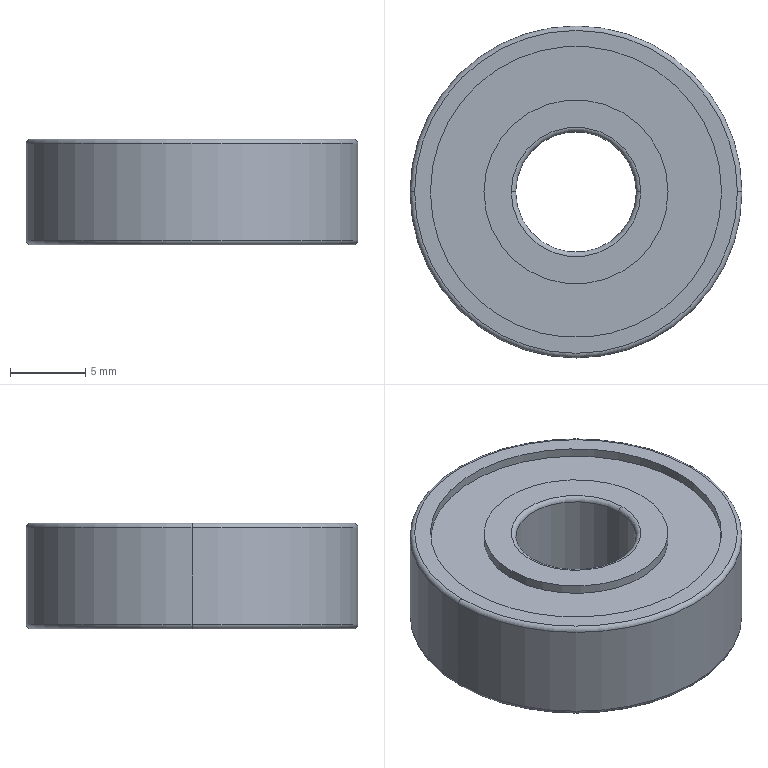Component | SolidWorks | JL001-05-02-1_B608ZZ-1 | 1 solid | 26 faces | box 22 x 22 x 7 mm | volume 2095 mm3 | cylinder 12 | torus 8 | plane 6 | commonest cylinder face diameters 12.2 x4 19.3 x4 22 x2 8 x2
build123d program:
from build123d import *


with BuildPart() as part:
    # Sketch1 → Revolve1 (revolve)
    with BuildSketch(Plane.XY, mode=Mode.PRIVATE) as revolve1_sk:
        with BuildLine():
            Line((0.3, 4), (6.7, 4))
            ThreePointArc((6.7, 4), (6.912, 4.088), (7, 4.3))
            Line((7, 4.3), (7, 6.1))
            Line((7, 6.1), (6.4, 6.1))
            Line((6.4, 6.1), (6.4, 9.65))
            Line((6.4, 9.65), (7, 9.65))
            Line((7, 9.65), (7, 10.7))
            ThreePointArc((7, 10.7), (6.912, 10.912), (6.7, 11))
            Line((6.7, 11), (0.3, 11))
            ThreePointArc((0.3, 11), (0.08787, 10.912), (0, 10.7))
            Line((0, 10.7), (0, 9.65))
            Line((0, 9.65), (0.6, 9.65))
            Line((0.6, 9.65), (0.6, 6.1))
            Line((0.6, 6.1), (0, 6.1))
            Line((0, 6.1), (0, 4.3))
            ThreePointArc((0, 4.3), (0.08787, 4.088), (0.3, 4))
        make_face()
    revolve(revolve1_sk.sketch.rotate(Axis((6.7, 0, 0), (-1, 0, 0)), 270), axis=Axis((6.7, 0, 0), (-1, 0, 0)))


solid = part.part

# Placed as in the assembly
solid = solid.moved(Location((0, 1047.5, 88), (0, 90, 0)))
STEP:
#1=COLOUR_RGB('',0.7922,0.8196,0.9333);
#2=FILL_AREA_STYLE_COLOUR('',#1);
#3=FILL_AREA_STYLE('',(#2));
#4=SURFACE_STYLE_FILL_AREA(#3);
#5=SURFACE_SIDE_STYLE('',(#4));
#6=SURFACE_STYLE_USAGE(.BOTH.,#5);
#7=PRESENTATION_STYLE_ASSIGNMENT((#6));
#8=CARTESIAN_POINT('',(-0.2402,41.24,3.441));
#9=VERTEX_POINT('',#8);
#10=CARTESIAN_POINT('',(0.2402,41.24,3.441));
#11=VERTEX_POINT('',#10);
#12=CARTESIAN_POINT('',(-0.,41.24,3.441));
#13=DIRECTION('',(0.,0.,1.));
#14=DIRECTION('',(-1.,0.,0.));
#15=AXIS2_PLACEMENT_3D('',#12,#13,#14);
#16=CIRCLE('',#15,0.2402);
#17=EDGE_CURVE('',#9,#11,#16,.T.);
#18=ORIENTED_EDGE('',*,*,#17,.T.);
#19=CARTESIAN_POINT('',(0.2402,41.24,3.465));
#20=VERTEX_POINT('',#19);
#21=CARTESIAN_POINT('',(0.2402,41.24,3.201));
#22=DIRECTION('',(0.,0.,1.));
#23=VECTOR('',#22,39.37);
#24=LINE('',#21,#23);
#25=EDGE_CURVE('',#11,#20,#24,.T.);
#26=ORIENTED_EDGE('',*,*,#25,.T.);
#27=CARTESIAN_POINT('',(-0.2402,41.24,3.465));
#28=VERTEX_POINT('',#27);
#29=CARTESIAN_POINT('',(-0.,41.24,3.465));
#30=DIRECTION('',(0.,0.,1.));
#31=DIRECTION('',(-1.,0.,0.));
#32=AXIS2_PLACEMENT_3D('',#29,#30,#31);
#33=CIRCLE('',#32,0.2402);
#34=EDGE_CURVE('',#28,#20,#33,.T.);
#35=ORIENTED_EDGE('',*,*,#34,.F.);
#36=CARTESIAN_POINT('',(-0.2402,41.24,3.201));
#37=DIRECTION('',(0.,0.,1.));
#38=VECTOR('',#37,39.37);
#39=LINE('',#36,#38);
#40=EDGE_CURVE('',#9,#28,#39,.T.);
#41=ORIENTED_EDGE('',*,*,#40,.F.);
#42=EDGE_LOOP('',(#18,#26,#35,#41));
#43=FACE_OUTER_BOUND('',#42,.T.);
#44=CARTESIAN_POINT('',(-0.,41.24,3.201));
#45=DIRECTION('',(0.,0.,1.));
#46=DIRECTION('',(-1.,0.,0.));
#47=AXIS2_PLACEMENT_3D('',#44,#45,#46);
#48=CYLINDRICAL_SURFACE('',#47,0.2402);
#49=ADVANCED_FACE('',(#43),#48,.T.);
#50=CARTESIAN_POINT('',(0.3799,41.24,3.441));
#51=VERTEX_POINT('',#50);
#52=CARTESIAN_POINT('',(-0.3799,41.24,3.441));
#53=VERTEX_POINT('',#52);
#54=CARTESIAN_POINT('',(-0.,41.24,3.441));
#55=DIRECTION('',(0.,0.,1.));
#56=DIRECTION('',(-1.,0.,0.));
#57=AXIS2_PLACEMENT_3D('',#54,#55,#56);
#58=CIRCLE('',#57,0.3799);
#59=EDGE_CURVE('',#51,#53,#58,.T.);
#60=ORIENTED_EDGE('',*,*,#59,.F.);
#61=CARTESIAN_POINT('',(0.3799,41.24,3.465));
#62=VERTEX_POINT('',#61);
#63=CARTESIAN_POINT('',(0.3799,41.24,3.201));
#64=DIRECTION('',(0.,0.,1.));
#65=VECTOR('',#64,39.37);
#66=LINE('',#63,#65);
#67=EDGE_CURVE('',#51,#62,#66,.T.);
#68=ORIENTED_EDGE('',*,*,#67,.T.);
#69=CARTESIAN_POINT('',(-0.3799,41.24,3.465));
#70=VERTEX_POINT('',#69);
#71=CARTESIAN_POINT('',(-0.,41.24,3.465));
#72=DIRECTION('',(0.,0.,1.));
#73=DIRECTION('',(-1.,0.,0.));
#74=AXIS2_PLACEMENT_3D('',#71,#72,#73);
#75=CIRCLE('',#74,0.3799);
#76=EDGE_CURVE('',#62,#70,#75,.T.);
#77=ORIENTED_EDGE('',*,*,#76,.T.);
#78=CARTESIAN_POINT('',(-0.3799,41.24,3.201));
#79=DIRECTION('',(0.,0.,1.));
#80=VECTOR('',#79,39.37);
#81=LINE('',#78,#80);
#82=EDGE_CURVE('',#53,#70,#81,.T.);
#83=ORIENTED_EDGE('',*,*,#82,.F.);
#84=EDGE_LOOP('',(#60,#68,#77,#83));
#85=FACE_OUTER_BOUND('',#84,.T.);
#86=CARTESIAN_POINT('',(-0.,41.24,3.201));
#87=DIRECTION('',(0.,0.,1.));
#88=DIRECTION('',(-1.,0.,0.));
#89=AXIS2_PLACEMENT_3D('',#86,#87,#88);
#90=CYLINDRICAL_SURFACE('',#89,0.3799);
#91=ADVANCED_FACE('',(#85),#90,.F.);
#92=CARTESIAN_POINT('',(-0.4331,41.24,3.453));
#93=VERTEX_POINT('',#92);
#94=CARTESIAN_POINT('',(0.4331,41.24,3.453));
#95=VERTEX_POINT('',#94);
#96=CARTESIAN_POINT('',(-0.,41.24,3.453));
#97=DIRECTION('',(0.,0.,1.));
#98=DIRECTION('',(-1.,0.,0.));
#99=AXIS2_PLACEMENT_3D('',#96,#97,#98);
#100=CIRCLE('',#99,0.4331);
#101=EDGE_CURVE('',#93,#95,#100,.T.);
#102=ORIENTED_EDGE('',*,*,#101,.T.);
#103=CARTESIAN_POINT('',(0.4213,41.24,3.465));
#104=VERTEX_POINT('',#103);
#105=CARTESIAN_POINT('',(0.4213,41.24,3.453));
#106=DIRECTION('',(-0.,-1.,0.));
#107=DIRECTION('',(1.,0.,0.));
#108=AXIS2_PLACEMENT_3D('',#105,#106,#107);
#109=CIRCLE('',#108,0.01181);
#110=EDGE_CURVE('',#95,#104,#109,.T.);
#111=ORIENTED_EDGE('',*,*,#110,.T.);
#112=CARTESIAN_POINT('',(-0.4213,41.24,3.465));
#113=VERTEX_POINT('',#112);
#114=CARTESIAN_POINT('',(-0.,41.24,3.465));
#115=DIRECTION('',(0.,0.,1.));
#116=DIRECTION('',(-1.,0.,0.));
#117=AXIS2_PLACEMENT_3D('',#114,#115,#116);
#118=CIRCLE('',#117,0.4213);
#119=EDGE_CURVE('',#113,#104,#118,.T.);
#120=ORIENTED_EDGE('',*,*,#119,.F.);
#121=CARTESIAN_POINT('',(-0.4213,41.24,3.453));
#122=DIRECTION('',(0.,1.,0.));
#123=DIRECTION('',(0.,0.,1.));
#124=AXIS2_PLACEMENT_3D('',#121,#122,#123);
#125=CIRCLE('',#124,0.01181);
#126=EDGE_CURVE('',#93,#113,#125,.T.);
#127=ORIENTED_EDGE('',*,*,#126,.F.);
#128=EDGE_LOOP('',(#102,#111,#120,#127));
#129=FACE_OUTER_BOUND('',#128,.T.);
#130=CARTESIAN_POINT('',(-0.,41.24,3.453));
#131=DIRECTION('',(0.,0.,1.));
#132=DIRECTION('',(-1.,0.,0.));
#133=AXIS2_PLACEMENT_3D('',#130,#131,#132);
#134=TOROIDAL_SURFACE('',#133,0.4213,0.01181);
#135=ADVANCED_FACE('',(#129),#134,.T.);
#136=CARTESIAN_POINT('',(-0.4331,41.24,3.201));
#137=VERTEX_POINT('',#136);
#138=CARTESIAN_POINT('',(0.4331,41.24,3.201));
#139=VERTEX_POINT('',#138);
#140=CARTESIAN_POINT('',(-0.,41.24,3.201));
#141=DIRECTION('',(0.,0.,1.));
#142=DIRECTION('',(-1.,0.,0.));
#143=AXIS2_PLACEMENT_3D('',#140,#141,#142);
#144=CIRCLE('',#143,0.4331);
#145=EDGE_CURVE('',#137,#139,#144,.T.);
#146=ORIENTED_EDGE('',*,*,#145,.T.);
#147=CARTESIAN_POINT('',(0.4331,41.24,3.201));
#148=DIRECTION('',(0.,0.,1.));
#149=VECTOR('',#148,39.37);
#150=LINE('',#147,#149);
#151=EDGE_CURVE('',#139,#95,#150,.T.);
#152=ORIENTED_EDGE('',*,*,#151,.T.);
#153=ORIENTED_EDGE('',*,*,#101,.F.);
#154=CARTESIAN_POINT('',(-0.4331,41.24,3.201));
#155=DIRECTION('',(0.,0.,1.));
#156=VECTOR('',#155,39.37);
#157=LINE('',#154,#156);
#158=EDGE_CURVE('',#137,#93,#157,.T.);
#159=ORIENTED_EDGE('',*,*,#158,.F.);
#160=EDGE_LOOP('',(#146,#152,#153,#159));
#161=FACE_OUTER_BOUND('',#160,.T.);
#162=CARTESIAN_POINT('',(-0.,41.24,3.201));
#163=DIRECTION('',(0.,0.,1.));
#164=DIRECTION('',(-1.,0.,0.));
#165=AXIS2_PLACEMENT_3D('',#162,#163,#164);
#166=CYLINDRICAL_SURFACE('',#165,0.4331);
#167=ADVANCED_FACE('',(#161),#166,.T.);
#168=CARTESIAN_POINT('',(-0.4213,41.24,3.189));
#169=VERTEX_POINT('',#168);
#170=CARTESIAN_POINT('',(0.4213,41.24,3.189));
#171=VERTEX_POINT('',#170);
#172=CARTESIAN_POINT('',(-0.,41.24,3.189));
#173=DIRECTION('',(0.,0.,1.));
#174=DIRECTION('',(-1.,0.,0.));
#175=AXIS2_PLACEMENT_3D('',#172,#173,#174);
#176=CIRCLE('',#175,0.4213);
#177=EDGE_CURVE('',#169,#171,#176,.T.);
#178=ORIENTED_EDGE('',*,*,#177,.T.);
#179=CARTESIAN_POINT('',(0.4213,41.24,3.201));
#180=DIRECTION('',(-0.,-1.,0.));
#181=DIRECTION('',(1.,0.,0.));
#182=AXIS2_PLACEMENT_3D('',#179,#180,#181);
#183=CIRCLE('',#182,0.01181);
#184=EDGE_CURVE('',#171,#139,#183,.T.);
#185=ORIENTED_EDGE('',*,*,#184,.T.);
#186=ORIENTED_EDGE('',*,*,#145,.F.);
#187=CARTESIAN_POINT('',(-0.4213,41.24,3.201));
#188=DIRECTION('',(0.,1.,0.));
#189=DIRECTION('',(0.,0.,1.));
#190=AXIS2_PLACEMENT_3D('',#187,#188,#189);
#191=CIRCLE('',#190,0.01181);
#192=EDGE_CURVE('',#169,#137,#191,.T.);
#193=ORIENTED_EDGE('',*,*,#192,.F.);
#194=EDGE_LOOP('',(#178,#185,#186,#193));
#195=FACE_OUTER_BOUND('',#194,.T.);
#196=CARTESIAN_POINT('',(-0.,41.24,3.201));
#197=DIRECTION('',(0.,0.,1.));
#198=DIRECTION('',(-1.,0.,0.));
#199=AXIS2_PLACEMENT_3D('',#196,#197,#198);
#200=TOROIDAL_SURFACE('',#199,0.4213,0.01181);
#201=ADVANCED_FACE('',(#195),#200,.T.);
#202=CARTESIAN_POINT('',(0.3799,41.24,3.189));
#203=VERTEX_POINT('',#202);
#204=CARTESIAN_POINT('',(-0.3799,41.24,3.189));
#205=VERTEX_POINT('',#204);
#206=CARTESIAN_POINT('',(-0.,41.24,3.189));
#207=DIRECTION('',(0.,0.,1.));
#208=DIRECTION('',(-1.,0.,0.));
#209=AXIS2_PLACEMENT_3D('',#206,#207,#208);
#210=CIRCLE('',#209,0.3799);
#211=EDGE_CURVE('',#203,#205,#210,.T.);
#212=ORIENTED_EDGE('',*,*,#211,.F.);
#213=CARTESIAN_POINT('',(0.3799,41.24,3.213));
#214=VERTEX_POINT('',#213);
#215=CARTESIAN_POINT('',(0.3799,41.24,3.201));
#216=DIRECTION('',(0.,0.,1.));
#217=VECTOR('',#216,39.37);
#218=LINE('',#215,#217);
#219=EDGE_CURVE('',#203,#214,#218,.T.);
#220=ORIENTED_EDGE('',*,*,#219,.T.);
#221=CARTESIAN_POINT('',(-0.3799,41.24,3.213));
#222=VERTEX_POINT('',#221);
#223=CARTESIAN_POINT('',(-0.,41.24,3.213));
#224=DIRECTION('',(0.,0.,1.));
#225=DIRECTION('',(-1.,0.,0.));
#226=AXIS2_PLACEMENT_3D('',#223,#224,#225);
#227=CIRCLE('',#226,0.3799);
#228=EDGE_CURVE('',#214,#222,#227,.T.);
#229=ORIENTED_EDGE('',*,*,#228,.T.);
#230=CARTESIAN_POINT('',(-0.3799,41.24,3.201));
#231=DIRECTION('',(0.,0.,1.));
#232=VECTOR('',#231,39.37);
#233=LINE('',#230,#232);
#234=EDGE_CURVE('',#205,#222,#233,.T.);
#235=ORIENTED_EDGE('',*,*,#234,.F.);
#236=EDGE_LOOP('',(#212,#220,#229,#235));
#237=FACE_OUTER_BOUND('',#236,.T.);
#238=CARTESIAN_POINT('',(-0.,41.24,3.201));
#239=DIRECTION('',(0.,0.,1.));
#240=DIRECTION('',(-1.,0.,0.));
#241=AXIS2_PLACEMENT_3D('',#238,#239,#240);
#242=CYLINDRICAL_SURFACE('',#241,0.3799);
#243=ADVANCED_FACE('',(#237),#242,.F.);
#244=CARTESIAN_POINT('',(-0.2402,41.24,3.189));
#245=VERTEX_POINT('',#244);
#246=CARTESIAN_POINT('',(0.2402,41.24,3.189));
#247=VERTEX_POINT('',#246);
#248=CARTESIAN_POINT('',(-0.,41.24,3.189));
#249=DIRECTION('',(0.,0.,1.));
#250=DIRECTION('',(-1.,0.,0.));
#251=AXIS2_PLACEMENT_3D('',#248,#249,#250);
#252=CIRCLE('',#251,0.2402);
#253=EDGE_CURVE('',#245,#247,#252,.T.);
#254=ORIENTED_EDGE('',*,*,#253,.T.);
#255=CARTESIAN_POINT('',(0.2402,41.24,3.213));
#256=VERTEX_POINT('',#255);
#257=CARTESIAN_POINT('',(0.2402,41.24,3.201));
#258=DIRECTION('',(0.,0.,1.));
#259=VECTOR('',#258,39.37);
#260=LINE('',#257,#259);
#261=EDGE_CURVE('',#247,#256,#260,.T.);
#262=ORIENTED_EDGE('',*,*,#261,.T.);
#263=CARTESIAN_POINT('',(-0.2402,41.24,3.213));
#264=VERTEX_POINT('',#263);
#265=CARTESIAN_POINT('',(-0.,41.24,3.213));
#266=DIRECTION('',(0.,0.,1.));
#267=DIRECTION('',(-1.,0.,0.));
#268=AXIS2_PLACEMENT_3D('',#265,#266,#267);
#269=CIRCLE('',#268,0.2402);
#270=EDGE_CURVE('',#264,#256,#269,.T.);
#271=ORIENTED_EDGE('',*,*,#270,.F.);
#272=CARTESIAN_POINT('',(-0.2402,41.24,3.201));
#273=DIRECTION('',(0.,0.,1.));
#274=VECTOR('',#273,39.37);
#275=LINE('',#272,#274);
#276=EDGE_CURVE('',#245,#264,#275,.T.);
#277=ORIENTED_EDGE('',*,*,#276,.F.);
#278=EDGE_LOOP('',(#254,#262,#271,#277));
#279=FACE_OUTER_BOUND('',#278,.T.);
#280=CARTESIAN_POINT('',(-0.,41.24,3.201));
#281=DIRECTION('',(0.,0.,1.));
#282=DIRECTION('',(-1.,0.,0.));
#283=AXIS2_PLACEMENT_3D('',#280,#281,#282);
#284=CYLINDRICAL_SURFACE('',#283,0.2402);
#285=ADVANCED_FACE('',(#279),#284,.T.);
#286=CARTESIAN_POINT('',(-0.1575,41.24,3.201));
#287=VERTEX_POINT('',#286);
#288=CARTESIAN_POINT('',(0.1575,41.24,3.201));
#289=VERTEX_POINT('',#288);
#290=CARTESIAN_POINT('',(-0.,41.24,3.201));
#291=DIRECTION('',(0.,0.,1.));
#292=DIRECTION('',(-1.,0.,0.));
#293=AXIS2_PLACEMENT_3D('',#290,#291,#292);
#294=CIRCLE('',#293,0.1575);
#295=EDGE_CURVE('',#287,#289,#294,.T.);
#296=ORIENTED_EDGE('',*,*,#295,.T.);
#297=CARTESIAN_POINT('',(0.1693,41.24,3.189));
#298=VERTEX_POINT('',#297);
#299=CARTESIAN_POINT('',(0.1693,41.24,3.201));
#300=DIRECTION('',(-0.,-1.,0.));
#301=DIRECTION('',(1.,0.,0.));
#302=AXIS2_PLACEMENT_3D('',#299,#300,#301);
#303=CIRCLE('',#302,0.01181);
#304=EDGE_CURVE('',#289,#298,#303,.T.);
#305=ORIENTED_EDGE('',*,*,#304,.T.);
#306=CARTESIAN_POINT('',(-0.1693,41.24,3.189));
#307=VERTEX_POINT('',#306);
#308=CARTESIAN_POINT('',(-0.,41.24,3.189));
#309=DIRECTION('',(0.,0.,1.));
#310=DIRECTION('',(-1.,0.,0.));
#311=AXIS2_PLACEMENT_3D('',#308,#309,#310);
#312=CIRCLE('',#311,0.1693);
#313=EDGE_CURVE('',#307,#298,#312,.T.);
#314=ORIENTED_EDGE('',*,*,#313,.F.);
#315=CARTESIAN_POINT('',(-0.1693,41.24,3.201));
#316=DIRECTION('',(0.,1.,0.));
#317=DIRECTION('',(0.,0.,1.));
#318=AXIS2_PLACEMENT_3D('',#315,#316,#317);
#319=CIRCLE('',#318,0.01181);
#320=EDGE_CURVE('',#287,#307,#319,.T.);
#321=ORIENTED_EDGE('',*,*,#320,.F.);
#322=EDGE_LOOP('',(#296,#305,#314,#321));
#323=FACE_OUTER_BOUND('',#322,.T.);
#324=CARTESIAN_POINT('',(-0.,41.24,3.201));
#325=DIRECTION('',(0.,0.,1.));
#326=DIRECTION('',(-1.,0.,0.));
#327=AXIS2_PLACEMENT_3D('',#324,#325,#326);
#328=TOROIDAL_SURFACE('',#327,0.1693,0.01181);
#329=ADVANCED_FACE('',(#323),#328,.T.);
#330=CARTESIAN_POINT('',(-0.,41.24,3.201));
#331=DIRECTION('',(0.,0.,1.));
#332=DIRECTION('',(-1.,0.,0.));
#333=AXIS2_PLACEMENT_3D('',#330,#331,#332);
#334=CIRCLE('',#333,0.1575);
#335=EDGE_CURVE('',#289,#287,#334,.T.);
#336=ORIENTED_EDGE('',*,*,#335,.F.);
#337=CARTESIAN_POINT('',(0.1575,41.24,3.453));
#338=VERTEX_POINT('',#337);
#339=CARTESIAN_POINT('',(0.1575,41.24,3.201));
#340=DIRECTION('',(0.,0.,1.));
#341=VECTOR('',#340,39.37);
#342=LINE('',#339,#341);
#343=EDGE_CURVE('',#289,#338,#342,.T.);
#344=ORIENTED_EDGE('',*,*,#343,.T.);
#345=CARTESIAN_POINT('',(-0.1575,41.24,3.453));
#346=VERTEX_POINT('',#345);
#347=CARTESIAN_POINT('',(-0.,41.24,3.453));
#348=DIRECTION('',(0.,0.,1.));
#349=DIRECTION('',(-1.,0.,0.));
#350=AXIS2_PLACEMENT_3D('',#347,#348,#349);
#351=CIRCLE('',#350,0.1575);
#352=EDGE_CURVE('',#338,#346,#351,.T.);
#353=ORIENTED_EDGE('',*,*,#352,.T.);
#354=CARTESIAN_POINT('',(-0.1575,41.24,3.201));
#355=DIRECTION('',(0.,0.,1.));
#356=VECTOR('',#355,39.37);
#357=LINE('',#354,#356);
#358=EDGE_CURVE('',#287,#346,#357,.T.);
#359=ORIENTED_EDGE('',*,*,#358,.F.);
#360=EDGE_LOOP('',(#336,#344,#353,#359));
#361=FACE_OUTER_BOUND('',#360,.T.);
#362=CARTESIAN_POINT('',(-0.,41.24,3.201));
#363=DIRECTION('',(0.,0.,1.));
#364=DIRECTION('',(-1.,0.,0.));
#365=AXIS2_PLACEMENT_3D('',#362,#363,#364);
#366=CYLINDRICAL_SURFACE('',#365,0.1575);
#367=ADVANCED_FACE('',(#361),#366,.F.);
#368=CARTESIAN_POINT('',(-0.1693,41.24,3.465));
#369=VERTEX_POINT('',#368);
#370=CARTESIAN_POINT('',(0.1693,41.24,3.465));
#371=VERTEX_POINT('',#370);
#372=CARTESIAN_POINT('',(-0.,41.24,3.465));
#373=DIRECTION('',(0.,0.,1.));
#374=DIRECTION('',(-1.,0.,0.));
#375=AXIS2_PLACEMENT_3D('',#372,#373,#374);
#376=CIRCLE('',#375,0.1693);
#377=EDGE_CURVE('',#369,#371,#376,.T.);
#378=ORIENTED_EDGE('',*,*,#377,.T.);
#379=CARTESIAN_POINT('',(0.1693,41.24,3.453));
#380=DIRECTION('',(-0.,-1.,0.));
#381=DIRECTION('',(1.,0.,0.));
#382=AXIS2_PLACEMENT_3D('',#379,#380,#381);
#383=CIRCLE('',#382,0.01181);
#384=EDGE_CURVE('',#371,#338,#383,.T.);
#385=ORIENTED_EDGE('',*,*,#384,.T.);
#386=CARTESIAN_POINT('',(-0.,41.24,3.453));
#387=DIRECTION('',(0.,0.,1.));
#388=DIRECTION('',(-1.,0.,0.));
#389=AXIS2_PLACEMENT_3D('',#386,#387,#388);
#390=CIRCLE('',#389,0.1575);
#391=EDGE_CURVE('',#346,#338,#390,.T.);
#392=ORIENTED_EDGE('',*,*,#391,.F.);
#393=CARTESIAN_POINT('',(-0.1693,41.24,3.453));
#394=DIRECTION('',(0.,1.,0.));
#395=DIRECTION('',(0.,0.,1.));
#396=AXIS2_PLACEMENT_3D('',#393,#394,#395);
#397=CIRCLE('',#396,0.01181);
#398=EDGE_CURVE('',#369,#346,#397,.T.);
#399=ORIENTED_EDGE('',*,*,#398,.F.);
#400=EDGE_LOOP('',(#378,#385,#392,#399));
#401=FACE_OUTER_BOUND('',#400,.T.);
#402=CARTESIAN_POINT('',(-0.,41.24,3.453));
#403=DIRECTION('',(0.,0.,1.));
#404=DIRECTION('',(-1.,0.,0.));
#405=AXIS2_PLACEMENT_3D('',#402,#403,#404);
#406=TOROIDAL_SURFACE('',#405,0.1693,0.01181);
#407=ADVANCED_FACE('',(#401),#406,.T.);
#408=ORIENTED_EDGE('',*,*,#384,.F.);
#409=CARTESIAN_POINT('',(-0.,41.24,3.465));
#410=DIRECTION('',(0.,0.,1.));
#411=DIRECTION('',(-1.,0.,0.));
#412=AXIS2_PLACEMENT_3D('',#409,#410,#411);
#413=CIRCLE('',#412,0.1693);
#414=EDGE_CURVE('',#371,#369,#413,.T.);
#415=ORIENTED_EDGE('',*,*,#414,.T.);
#416=ORIENTED_EDGE('',*,*,#398,.T.);
#417=ORIENTED_EDGE('',*,*,#352,.F.);
#418=EDGE_LOOP('',(#408,#415,#416,#417));
#419=FACE_OUTER_BOUND('',#418,.T.);
#420=CARTESIAN_POINT('',(-0.,41.24,3.453));
#421=DIRECTION('',(0.,0.,1.));
#422=DIRECTION('',(-1.,0.,0.));
#423=AXIS2_PLACEMENT_3D('',#420,#421,#422);
#424=TOROIDAL_SURFACE('',#423,0.1693,0.01181);
#425=ADVANCED_FACE('',(#419),#424,.T.);
#426=ORIENTED_EDGE('',*,*,#343,.F.);
#427=ORIENTED_EDGE('',*,*,#295,.F.);
#428=ORIENTED_EDGE('',*,*,#358,.T.);
#429=ORIENTED_EDGE('',*,*,#391,.T.);
#430=EDGE_LOOP('',(#426,#427,#428,#429));
#431=FACE_OUTER_BOUND('',#430,.T.);
#432=CARTESIAN_POINT('',(-0.,41.24,3.201));
#433=DIRECTION('',(0.,0.,1.));
#434=DIRECTION('',(-1.,0.,0.));
#435=AXIS2_PLACEMENT_3D('',#432,#433,#434);
#436=CYLINDRICAL_SURFACE('',#435,0.1575);
#437=ADVANCED_FACE('',(#431),#436,.F.);
#438=ORIENTED_EDGE('',*,*,#304,.F.);
#439=ORIENTED_EDGE('',*,*,#335,.T.);
#440=ORIENTED_EDGE('',*,*,#320,.T.);
#441=CARTESIAN_POINT('',(-0.,41.24,3.189));
#442=DIRECTION('',(0.,0.,1.));
#443=DIRECTION('',(-1.,0.,0.));
#444=AXIS2_PLACEMENT_3D('',#441,#442,#443);
#445=CIRCLE('',#444,0.1693);
#446=EDGE_CURVE('',#298,#307,#445,.T.);
#447=ORIENTED_EDGE('',*,*,#446,.F.);
#448=EDGE_LOOP('',(#438,#439,#440,#447));
#449=FACE_OUTER_BOUND('',#448,.T.);
#450=CARTESIAN_POINT('',(-0.,41.24,3.201));
#451=DIRECTION('',(0.,0.,1.));
#452=DIRECTION('',(-1.,0.,0.));
#453=AXIS2_PLACEMENT_3D('',#450,#451,#452);
#454=TOROIDAL_SURFACE('',#453,0.1693,0.01181);
#455=ADVANCED_FACE('',(#449),#454,.T.);
#456=ORIENTED_EDGE('',*,*,#253,.F.);
#457=CARTESIAN_POINT('',(-0.,41.24,3.189));
#458=DIRECTION('',(0.,0.,1.));
#459=DIRECTION('',(-1.,0.,0.));
#460=AXIS2_PLACEMENT_3D('',#457,#458,#459);
#461=CIRCLE('',#460,0.2402);
#462=EDGE_CURVE('',#247,#245,#461,.T.);
#463=ORIENTED_EDGE('',*,*,#462,.F.);
#464=EDGE_LOOP('',(#456,#463));
#465=FACE_OUTER_BOUND('',#464,.T.);
#466=ORIENTED_EDGE('',*,*,#313,.T.);
#467=ORIENTED_EDGE('',*,*,#446,.T.);
#468=EDGE_LOOP('',(#466,#467));
#469=FACE_BOUND('',#468,.T.);
#470=CARTESIAN_POINT('',(-0.,41.071,3.189));
#471=DIRECTION('',(0.,0.,1.));
#472=DIRECTION('',(-1.,0.,0.));
#473=AXIS2_PLACEMENT_3D('',#470,#471,#472);
#474=PLANE('',#473);
#475=ADVANCED_FACE('',(#465,#469),#474,.F.);
#476=ORIENTED_EDGE('',*,*,#261,.F.);
#477=ORIENTED_EDGE('',*,*,#462,.T.);
#478=ORIENTED_EDGE('',*,*,#276,.T.);
#479=CARTESIAN_POINT('',(-0.,41.24,3.213));
#480=DIRECTION('',(0.,0.,1.));
#481=DIRECTION('',(-1.,0.,0.));
#482=AXIS2_PLACEMENT_3D('',#479,#480,#481);
#483=CIRCLE('',#482,0.2402);
#484=EDGE_CURVE('',#256,#264,#483,.T.);
#485=ORIENTED_EDGE('',*,*,#484,.F.);
#486=EDGE_LOOP('',(#476,#477,#478,#485));
#487=FACE_OUTER_BOUND('',#486,.T.);
#488=CARTESIAN_POINT('',(-0.,41.24,3.201));
#489=DIRECTION('',(0.,0.,1.));
#490=DIRECTION('',(-1.,0.,0.));
#491=AXIS2_PLACEMENT_3D('',#488,#489,#490);
#492=CYLINDRICAL_SURFACE('',#491,0.2402);
#493=ADVANCED_FACE('',(#487),#492,.T.);
#494=CARTESIAN_POINT('',(-0.,41.24,3.213));
#495=DIRECTION('',(0.,0.,1.));
#496=DIRECTION('',(-1.,0.,0.));
#497=AXIS2_PLACEMENT_3D('',#494,#495,#496);
#498=CIRCLE('',#497,0.3799);
#499=EDGE_CURVE('',#222,#214,#498,.T.);
#500=ORIENTED_EDGE('',*,*,#499,.F.);
#501=ORIENTED_EDGE('',*,*,#228,.F.);
#502=EDGE_LOOP('',(#500,#501));
#503=FACE_OUTER_BOUND('',#502,.T.);
#504=ORIENTED_EDGE('',*,*,#270,.T.);
#505=ORIENTED_EDGE('',*,*,#484,.T.);
#506=EDGE_LOOP('',(#504,#505));
#507=FACE_BOUND('',#506,.T.);
#508=CARTESIAN_POINT('',(-0.,41.,3.213));
#509=DIRECTION('',(0.,0.,1.));
#510=DIRECTION('',(-1.,0.,0.));
#511=AXIS2_PLACEMENT_3D('',#508,#509,#510);
#512=PLANE('',#511);
#513=ADVANCED_FACE('',(#503,#507),#512,.F.);
#514=ORIENTED_EDGE('',*,*,#219,.F.);
#515=CARTESIAN_POINT('',(-0.,41.24,3.189));
#516=DIRECTION('',(0.,0.,1.));
#517=DIRECTION('',(-1.,0.,0.));
#518=AXIS2_PLACEMENT_3D('',#515,#516,#517);
#519=CIRCLE('',#518,0.3799);
#520=EDGE_CURVE('',#205,#203,#519,.T.);
#521=ORIENTED_EDGE('',*,*,#520,.F.);
#522=ORIENTED_EDGE('',*,*,#234,.T.);
#523=ORIENTED_EDGE('',*,*,#499,.T.);
#524=EDGE_LOOP('',(#514,#521,#522,#523));
#525=FACE_OUTER_BOUND('',#524,.T.);
#526=CARTESIAN_POINT('',(-0.,41.24,3.201));
#527=DIRECTION('',(0.,0.,1.));
#528=DIRECTION('',(-1.,0.,0.));
#529=AXIS2_PLACEMENT_3D('',#526,#527,#528);
#530=CYLINDRICAL_SURFACE('',#529,0.3799);
#531=ADVANCED_FACE('',(#525),#530,.F.);
#532=ORIENTED_EDGE('',*,*,#177,.F.);
#533=CARTESIAN_POINT('',(-0.,41.24,3.189));
#534=DIRECTION('',(0.,0.,1.));
#535=DIRECTION('',(-1.,0.,0.));
#536=AXIS2_PLACEMENT_3D('',#533,#534,#535);
#537=CIRCLE('',#536,0.4213);
#538=EDGE_CURVE('',#171,#169,#537,.T.);
#539=ORIENTED_EDGE('',*,*,#538,.F.);
#540=EDGE_LOOP('',(#532,#539));
#541=FACE_OUTER_BOUND('',#540,.T.);
#542=ORIENTED_EDGE('',*,*,#520,.T.);
#543=ORIENTED_EDGE('',*,*,#211,.T.);
#544=EDGE_LOOP('',(#542,#543));
#545=FACE_BOUND('',#544,.T.);
#546=CARTESIAN_POINT('',(-0.,40.86,3.189));
#547=DIRECTION('',(0.,0.,1.));
#548=DIRECTION('',(-1.,0.,0.));
#549=AXIS2_PLACEMENT_3D('',#546,#547,#548);
#550=PLANE('',#549);
#551=ADVANCED_FACE('',(#541,#545),#550,.F.);
#552=ORIENTED_EDGE('',*,*,#184,.F.);
#553=ORIENTED_EDGE('',*,*,#538,.T.);
#554=ORIENTED_EDGE('',*,*,#192,.T.);
#555=CARTESIAN_POINT('',(-0.,41.24,3.201));
#556=DIRECTION('',(0.,0.,1.));
#557=DIRECTION('',(-1.,0.,0.));
#558=AXIS2_PLACEMENT_3D('',#555,#556,#557);
#559=CIRCLE('',#558,0.4331);
#560=EDGE_CURVE('',#139,#137,#559,.T.);
#561=ORIENTED_EDGE('',*,*,#560,.F.);
#562=EDGE_LOOP('',(#552,#553,#554,#561));
#563=FACE_OUTER_BOUND('',#562,.T.);
#564=CARTESIAN_POINT('',(-0.,41.24,3.201));
#565=DIRECTION('',(0.,0.,1.));
#566=DIRECTION('',(-1.,0.,0.));
#567=AXIS2_PLACEMENT_3D('',#564,#565,#566);
#568=TOROIDAL_SURFACE('',#567,0.4213,0.01181);
#569=ADVANCED_FACE('',(#563),#568,.T.);
#570=ORIENTED_EDGE('',*,*,#151,.F.);
#571=ORIENTED_EDGE('',*,*,#560,.T.);
#572=ORIENTED_EDGE('',*,*,#158,.T.);
#573=CARTESIAN_POINT('',(-0.,41.24,3.453));
#574=DIRECTION('',(0.,0.,1.));
#575=DIRECTION('',(-1.,0.,0.));
#576=AXIS2_PLACEMENT_3D('',#573,#574,#575);
#577=CIRCLE('',#576,0.4331);
#578=EDGE_CURVE('',#95,#93,#577,.T.);
#579=ORIENTED_EDGE('',*,*,#578,.F.);
#580=EDGE_LOOP('',(#570,#571,#572,#579));
#581=FACE_OUTER_BOUND('',#580,.T.);
#582=CARTESIAN_POINT('',(-0.,41.24,3.201));
#583=DIRECTION('',(0.,0.,1.));
#584=DIRECTION('',(-1.,0.,0.));
#585=AXIS2_PLACEMENT_3D('',#582,#583,#584);
#586=CYLINDRICAL_SURFACE('',#585,0.4331);
#587=ADVANCED_FACE('',(#581),#586,.T.);
#588=ORIENTED_EDGE('',*,*,#110,.F.);
#589=ORIENTED_EDGE('',*,*,#578,.T.);
#590=ORIENTED_EDGE('',*,*,#126,.T.);
#591=CARTESIAN_POINT('',(-0.,41.24,3.465));
#592=DIRECTION('',(0.,0.,1.));
#593=DIRECTION('',(-1.,0.,0.));
#594=AXIS2_PLACEMENT_3D('',#591,#592,#593);
#595=CIRCLE('',#594,0.4213);
#596=EDGE_CURVE('',#104,#113,#595,.T.);
#597=ORIENTED_EDGE('',*,*,#596,.F.);
#598=EDGE_LOOP('',(#588,#589,#590,#597));
#599=FACE_OUTER_BOUND('',#598,.T.);
#600=CARTESIAN_POINT('',(-0.,41.24,3.453));
#601=DIRECTION('',(0.,0.,1.));
#602=DIRECTION('',(-1.,0.,0.));
#603=AXIS2_PLACEMENT_3D('',#600,#601,#602);
#604=TOROIDAL_SURFACE('',#603,0.4213,0.01181);
#605=ADVANCED_FACE('',(#599),#604,.T.);
#606=CARTESIAN_POINT('',(-0.,41.24,3.465));
#607=DIRECTION('',(0.,0.,1.));
#608=DIRECTION('',(-1.,0.,0.));
#609=AXIS2_PLACEMENT_3D('',#606,#607,#608);
#610=CIRCLE('',#609,0.3799);
#611=EDGE_CURVE('',#70,#62,#610,.T.);
#612=ORIENTED_EDGE('',*,*,#611,.F.);
#613=ORIENTED_EDGE('',*,*,#76,.F.);
#614=EDGE_LOOP('',(#612,#613));
#615=FACE_BOUND('',#614,.T.);
#616=ORIENTED_EDGE('',*,*,#119,.T.);
#617=ORIENTED_EDGE('',*,*,#596,.T.);
#618=EDGE_LOOP('',(#616,#617));
#619=FACE_OUTER_BOUND('',#618,.T.);
#620=CARTESIAN_POINT('',(-0.,40.819,3.465));
#621=DIRECTION('',(-0.,0.,-1.));
#622=DIRECTION('',(1.,0.,-0.));
#623=AXIS2_PLACEMENT_3D('',#620,#621,#622);
#624=PLANE('',#623);
#625=ADVANCED_FACE('',(#615,#619),#624,.F.);
#626=ORIENTED_EDGE('',*,*,#67,.F.);
#627=CARTESIAN_POINT('',(-0.,41.24,3.441));
#628=DIRECTION('',(0.,0.,1.));
#629=DIRECTION('',(-1.,0.,0.));
#630=AXIS2_PLACEMENT_3D('',#627,#628,#629);
#631=CIRCLE('',#630,0.3799);
#632=EDGE_CURVE('',#53,#51,#631,.T.);
#633=ORIENTED_EDGE('',*,*,#632,.F.);
#634=ORIENTED_EDGE('',*,*,#82,.T.);
#635=ORIENTED_EDGE('',*,*,#611,.T.);
#636=EDGE_LOOP('',(#626,#633,#634,#635));
#637=FACE_OUTER_BOUND('',#636,.T.);
#638=CARTESIAN_POINT('',(-0.,41.24,3.201));
#639=DIRECTION('',(0.,0.,1.));
#640=DIRECTION('',(-1.,0.,0.));
#641=AXIS2_PLACEMENT_3D('',#638,#639,#640);
#642=CYLINDRICAL_SURFACE('',#641,0.3799);
#643=ADVANCED_FACE('',(#637),#642,.F.);
#644=ORIENTED_EDGE('',*,*,#17,.F.);
#645=CARTESIAN_POINT('',(-0.,41.24,3.441));
#646=DIRECTION('',(0.,0.,1.));
#647=DIRECTION('',(-1.,0.,0.));
#648=AXIS2_PLACEMENT_3D('',#645,#646,#647);
#649=CIRCLE('',#648,0.2402);
#650=EDGE_CURVE('',#11,#9,#649,.T.);
#651=ORIENTED_EDGE('',*,*,#650,.F.);
#652=EDGE_LOOP('',(#644,#651));
#653=FACE_BOUND('',#652,.T.);
#654=ORIENTED_EDGE('',*,*,#632,.T.);
#655=ORIENTED_EDGE('',*,*,#59,.T.);
#656=EDGE_LOOP('',(#654,#655));
#657=FACE_OUTER_BOUND('',#656,.T.);
#658=CARTESIAN_POINT('',(-0.,40.86,3.441));
#659=DIRECTION('',(-0.,0.,-1.));
#660=DIRECTION('',(1.,0.,-0.));
#661=AXIS2_PLACEMENT_3D('',#658,#659,#660);
#662=PLANE('',#661);
#663=ADVANCED_FACE('',(#653,#657),#662,.F.);
#664=ORIENTED_EDGE('',*,*,#25,.F.);
#665=ORIENTED_EDGE('',*,*,#650,.T.);
#666=ORIENTED_EDGE('',*,*,#40,.T.);
#667=CARTESIAN_POINT('',(-0.,41.24,3.465));
#668=DIRECTION('',(0.,0.,1.));
#669=DIRECTION('',(-1.,0.,0.));
#670=AXIS2_PLACEMENT_3D('',#667,#668,#669);
#671=CIRCLE('',#670,0.2402);
#672=EDGE_CURVE('',#20,#28,#671,.T.);
#673=ORIENTED_EDGE('',*,*,#672,.F.);
#674=EDGE_LOOP('',(#664,#665,#666,#673));
#675=FACE_OUTER_BOUND('',#674,.T.);
#676=CARTESIAN_POINT('',(-0.,41.24,3.201));
#677=DIRECTION('',(0.,0.,1.));
#678=DIRECTION('',(-1.,0.,0.));
#679=AXIS2_PLACEMENT_3D('',#676,#677,#678);
#680=CYLINDRICAL_SURFACE('',#679,0.2402);
#681=ADVANCED_FACE('',(#675),#680,.T.);
#682=ORIENTED_EDGE('',*,*,#377,.F.);
#683=ORIENTED_EDGE('',*,*,#414,.F.);
#684=EDGE_LOOP('',(#682,#683));
#685=FACE_BOUND('',#684,.T.);
#686=ORIENTED_EDGE('',*,*,#34,.T.);
#687=ORIENTED_EDGE('',*,*,#672,.T.);
#688=EDGE_LOOP('',(#686,#687));
#689=FACE_OUTER_BOUND('',#688,.T.);
#690=CARTESIAN_POINT('',(-0.,41.,3.465));
#691=DIRECTION('',(-0.,0.,-1.));
#692=DIRECTION('',(1.,0.,-0.));
#693=AXIS2_PLACEMENT_3D('',#690,#691,#692);
#694=PLANE('',#693);
#695=ADVANCED_FACE('',(#685,#689),#694,.F.);
#696=CLOSED_SHELL('',(#49,#91,#135,#167,#201,#243,#285,#329,#367,#407,#425,#437,#455,#475,#493,#513,#531,#551,#569,#587,#605,#625,#643,#663,#681,#695));
#697=MANIFOLD_SOLID_BREP('',#696);
#698=STYLED_ITEM('',(#7),#697);
#699=PRESENTATION_LAYER_ASSIGNMENT('','',(#698));
#700=CARTESIAN_POINT('',(0.,0.,0.));
#701=DIRECTION('',(0.,0.,1.));
#702=DIRECTION('',(1.,0.,0.));
#703=AXIS2_PLACEMENT_3D('',#700,#701,#702);
#704=(LENGTH_UNIT()NAMED_UNIT(*)SI_UNIT($,.METRE.));
#705=LENGTH_MEASURE_WITH_UNIT(LENGTH_MEASURE(0.0254),#704);
#706=DIMENSIONAL_EXPONENTS(1.,0.,0.,0.,0.,0.,0.);
#707=(CONVERSION_BASED_UNIT('',#705)LENGTH_UNIT()NAMED_UNIT(#706));
#708=UNCERTAINTY_MEASURE_WITH_UNIT(LENGTH_MEASURE(0.00001),#707,'','');
#709=(NAMED_UNIT(*)PLANE_ANGLE_UNIT()SI_UNIT($,.RADIAN.));
#710=(NAMED_UNIT(*)SI_UNIT($,.STERADIAN.)SOLID_ANGLE_UNIT());
#711=(GEOMETRIC_REPRESENTATION_CONTEXT(3)GLOBAL_UNCERTAINTY_ASSIGNED_CONTEXT((#708))GLOBAL_UNIT_ASSIGNED_CONTEXT((#707,#709,#710))REPRESENTATION_CONTEXT('',''));
#712=ADVANCED_BREP_SHAPE_REPRESENTATION('',(#697,#703),#711);
#713=(LENGTH_UNIT()NAMED_UNIT(*)SI_UNIT($,.METRE.));
#714=LENGTH_MEASURE_WITH_UNIT(LENGTH_MEASURE(0.0254),#713);
#715=DIMENSIONAL_EXPONENTS(1.,0.,0.,0.,0.,0.,0.);
#716=(CONVERSION_BASED_UNIT('',#714)LENGTH_UNIT()NAMED_UNIT(#715));
#717=UNCERTAINTY_MEASURE_WITH_UNIT(LENGTH_MEASURE(0.00001),#716,'','');
#718=(NAMED_UNIT(*)PLANE_ANGLE_UNIT()SI_UNIT($,.RADIAN.));
#719=(NAMED_UNIT(*)SI_UNIT($,.STERADIAN.)SOLID_ANGLE_UNIT());
#720=(GEOMETRIC_REPRESENTATION_CONTEXT(3)GLOBAL_UNCERTAINTY_ASSIGNED_CONTEXT((#717))GLOBAL_UNIT_ASSIGNED_CONTEXT((#716,#718,#719))REPRESENTATION_CONTEXT('',''));
#721=MECHANICAL_DESIGN_GEOMETRIC_PRESENTATION_REPRESENTATION('',(#698),#720);